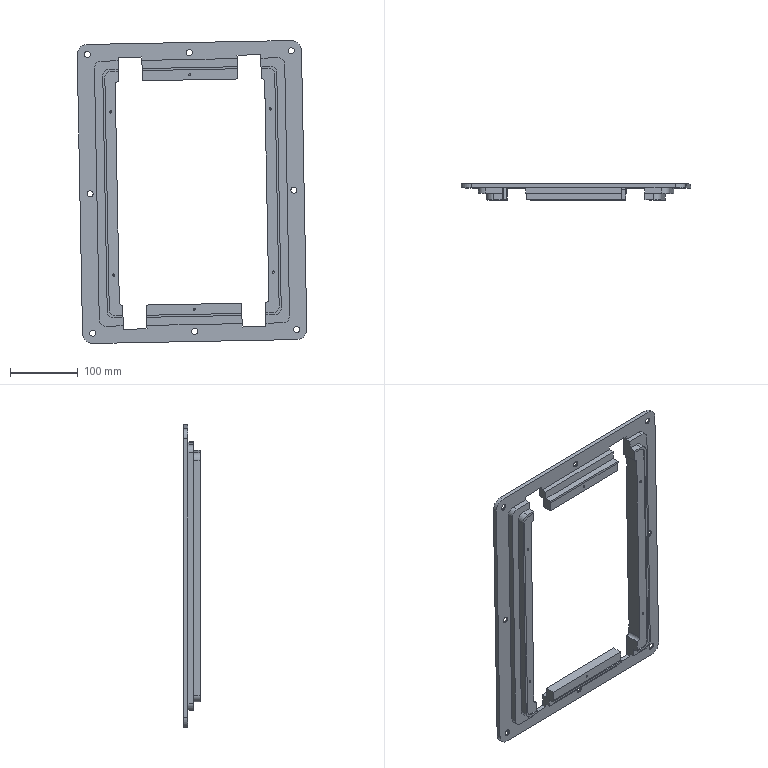Component | SolidWorks | 15BrushPlateThickInnerFrameOneOutOfTwo-1 | 1 solid | 141 faces | box 337.75 x 24 x 445.64 mm | volume 782663 mm3 | plane 63 | cylinder 50 | cone 28 | commonest cylinder face diameters 9 x16 3.3 x12 20 x12 10 x4 30 x4 12.125 x2 | material A3 Steel
build123d program:
from build123d import *

# Parameters (mm, degrees)
BOSS_EXTRUDE1_DEPTH                                  = 6
BOSS_EXTRUDE2_DEPTH                                  = 18
CUT_EXTRUDE1_DEPTH                                   = 277.045
CUT_EXTRUDE2_DEPTH                                   = 1.5
HOLE_SIZE_ACCORDING_TO_TYPE_OF_HEXAGON_S_D           = 9
HOLE_SIZE_ACCORDING_TO_TYPE_OF_HEXAGON_S_CSINK_D     = 17.6
HOLE_SIZE_ACCORDING_TO_TYPE_OF_HEXAGON_S_CSINK_ANGLE = 90
M4_TAPPED_HOLE1_D                                    = 3.3
M4_TAPPED_HOLE1_DEPTH                                = 8.1
M4_TAPPED_HOLE1_TIP                                  = 0.9914
CUT_EXTRUDE3_START                                   = -10
CUT_EXTRUDE3_DEPTH                                   = 10
SKETCH13_W                                           = 35
SKETCH13_H                                           = 35
CUT_EXTRUDE4_DEPTH                                   = 277.045
MIRROR2_COPY_1_SKETCH_W                              = 35
MIRROR2_COPY_1_SKETCH_H                              = 35
MIRROR2_COPY_1_DEPTH                                 = 277.045
SKETCH14_W                                           = 16
SKETCH14_H                                           = 140
CUT_EXTRUDE5_DEPTH                                   = 8
CUT_EXTRUDE6_REACH                                   = 399.336
SKETCH15_R                                           = 6.062


with BuildPart() as part:
    # Sketch1 → Boss-Extrude1 (new body)
    with BuildSketch(Plane.XY):
        with BuildLine():
            Line((-205, -165), (205, -165))
            ThreePointArc((205, -165), (215.607, -160.607), (220, -150))
            Line((220, -150), (220, 150))
            ThreePointArc((220, 150), (215.607, 160.607), (205, 165))
            Line((205, 165), (-205, 165))
            ThreePointArc((-205, 165), (-215.607, 160.607), (-220, 150))
            Line((-220, 150), (-220, -150))
            ThreePointArc((-220, -150), (-215.607, -160.607), (-205, -165))
        make_face()
    extrude(amount=-BOSS_EXTRUDE1_DEPTH)

    # Sketch2 → Boss-Extrude2 (add)
    with BuildSketch(Plane(origin=(0, 0, -6), x_dir=(-1, 0, 0), z_dir=(0, 0, -1))):
        with BuildLine():
            Line((-185, -140), (185, -140))
            ThreePointArc((185, -140), (192.071, -137.071), (195, -130))
            Line((195, -130), (195, 130))
            ThreePointArc((195, 130), (192.071, 137.071), (185, 140))
            Line((185, 140), (-185, 140))
            ThreePointArc((-185, 140), (-192.071, 137.071), (-195, 130))
            Line((-195, 130), (-195, -130))
            ThreePointArc((-195, -130), (-192.071, -137.071), (-185, -140))
        make_face()
    extrude(amount=BOSS_EXTRUDE2_DEPTH)

    # Sketch3 → Cut-Extrude1 (cut, through all)
    with BuildSketch(Plane.XY):
        with BuildLine():
            Line((-160, -110), (160, -110))
            ThreePointArc((160, -110), (163.536, -108.536), (165, -105))
            Line((165, -105), (165, 105))
            ThreePointArc((165, 105), (163.536, 108.536), (160, 110))
            Line((160, 110), (-160, 110))
            ThreePointArc((-160, 110), (-163.536, 108.536), (-165, 105))
            Line((-165, 105), (-165, -105))
            ThreePointArc((-165, -105), (-163.536, -108.536), (-160, -110))
        make_face()
    extrude(amount=-CUT_EXTRUDE1_DEPTH, mode=Mode.SUBTRACT)

    # Sketch4 → Cut-Extrude2 (cut)
    with BuildSketch(Plane.XY.offset(-24)):
        with BuildLine():
            Line((-170, -125), (170, -125))
            ThreePointArc((170, -125), (177.071, -122.071), (180, -115))
            Line((180, -115), (180, 115))
            ThreePointArc((180, 115), (177.071, 122.071), (170, 125))
            Line((170, 125), (-170, 125))
            ThreePointArc((-170, 125), (-177.071, 122.071), (-180, 115))
            Line((-180, 115), (-180, -115))
            ThreePointArc((-180, -115), (-177.071, -122.071), (-170, -125))
        make_face()
    extrude(amount=CUT_EXTRUDE2_DEPTH, mode=Mode.SUBTRACT)

    # Hole Size_According to_Type of Hexagon S (through all)
    with Locations(Plane(origin=(-205, 150, 0), x_dir=(1, 0, 0), z_dir=(0, 0, 1))):
        with Locations((0, 0), (0, -300), (410, -300), (410, 0), (410, -150), (205, 0), (0, -150), (205, -300)):
            CounterSinkHole(HOLE_SIZE_ACCORDING_TO_TYPE_OF_HEXAGON_S_D / 2, HOLE_SIZE_ACCORDING_TO_TYPE_OF_HEXAGON_S_CSINK_D / 2, counter_sink_angle=HOLE_SIZE_ACCORDING_TO_TYPE_OF_HEXAGON_S_CSINK_ANGLE)

    # M4 Tapped Hole1
    with Locations(Plane(origin=(172.5, 0, -22.5), x_dir=(-1, 0, 0), z_dir=(0, 0, -1))):
        with Locations((0, 0), (345, 0), (292.5, 117.5), (52.5, 117.5), (292.5, -117.5), (52.5, -117.5)):
            Hole(M4_TAPPED_HOLE1_D / 2, depth=M4_TAPPED_HOLE1_DEPTH)
            with Locations((0, 0, -(M4_TAPPED_HOLE1_DEPTH + M4_TAPPED_HOLE1_TIP / 2))):  # 118° drill point
                Cone(0, M4_TAPPED_HOLE1_D / 2, M4_TAPPED_HOLE1_TIP, mode=Mode.SUBTRACT)

    # Sketch12 → Cut-Extrude3 (cut)
    with BuildSketch(Plane(origin=(0, 0, -24), x_dir=(-1, 0, 0), z_dir=(0, 0, -1)).offset(CUT_EXTRUDE3_START)):
        with BuildLine():
            Line((185, 140), (-185, 140))
            ThreePointArc((-185, 140), (-192.071, 137.071), (-195, 130))
            Line((-195, 130), (-195, -130))
            ThreePointArc((-195, -130), (-192.071, -137.071), (-185, -140))
            Line((-185, -140), (185, -140))
            ThreePointArc((185, -140), (192.071, -137.071), (195, -130))
            Line((195, -130), (195, 130))
            ThreePointArc((195, 130), (192.071, 137.071), (185, 140))
        make_face()
        with BuildLine():
            Line((-173, -128), (173, -128))
            ThreePointArc((173, -128), (180.071, -125.071), (183, -118))
            Line((183, -118), (183, 118))
            ThreePointArc((183, 118), (180.071, 125.071), (173, 128))
            Line((173, 128), (-173, 128))
            ThreePointArc((-173, 128), (-180.071, 125.071), (-183, 118))
            Line((-183, 118), (-183, -118))
            ThreePointArc((-183, -118), (-180.071, -125.071), (-173, -128))
        make_face(mode=Mode.SUBTRACT)
    extrude(amount=CUT_EXTRUDE3_DEPTH, mode=Mode.SUBTRACT)

    # Sketch13 → Cut-Extrude4 (cut, through all)
    with BuildSketch(Plane.XY):
        with Locations((-182.5, 87.5)):
            Rectangle(SKETCH13_W, SKETCH13_H)
    cut_extrude4 = extrude(amount=-CUT_EXTRUDE4_DEPTH, mode=Mode.SUBTRACT)

    # Mirror1: Cut-Extrude4 across plane
    add(cut_extrude4.mirror(Plane.ZX), mode=Mode.SUBTRACT)

    # Mirror2: Cut-Extrude4 across plane
    add(cut_extrude4.mirror(Plane(origin=(0, 0, 0), x_dir=(0, 0, 1), z_dir=(1, 0, 0))), mode=Mode.SUBTRACT)

    # Mirror2 copy 1 sketch → Mirror2 copy 1 (cut, through all)
    with BuildSketch(Plane(origin=(0, 0, 0), x_dir=(-1, 0, 0), z_dir=(0, 0, 1))):
        with Locations((-182.5, 87.5)):
            Rectangle(MIRROR2_COPY_1_SKETCH_W, MIRROR2_COPY_1_SKETCH_H)
    extrude(amount=-MIRROR2_COPY_1_DEPTH, mode=Mode.SUBTRACT)

    # Sketch14 → Cut-Extrude5 (cut)
    with BuildSketch(Plane.XY):
        with Locations((-173, 0)):
            Rectangle(SKETCH14_W, SKETCH14_H)
    cut_extrude5 = extrude(amount=-CUT_EXTRUDE5_DEPTH, mode=Mode.SUBTRACT)

    # Mirror3: Cut-Extrude5 across plane
    add(cut_extrude5.mirror(Plane(origin=(0, 0, 0), x_dir=(0, 0, 1), z_dir=(1, 0, 0))), mode=Mode.SUBTRACT)

    # Sketch15 → Cut-Extrude6 (cut, up to next)
    with BuildSketch(Plane(origin=(0, 165, 0), x_dir=(1, 0, 0), z_dir=(0, 1, 0)), mode=Mode.PRIVATE) as cut_extrude6_sk1:
        with Locations((-143.5, -4.062)):
            Circle(SKETCH15_R)
    cut_extrude6_tool1 = extrude(cut_extrude6_sk1.sketch, amount=-CUT_EXTRUDE6_REACH, mode=Mode.PRIVATE) & part.part
    cut_extrude6 = cut_extrude6_tool1.solids().sort_by_distance((-143.5, 165, 4.062))[0]
    add(cut_extrude6, mode=Mode.SUBTRACT)

    # Mirror4: Cut-Extrude6 across plane
    add(cut_extrude6.mirror(Plane(origin=(0, 0, 0), x_dir=(0, 0, 1), z_dir=(1, 0, 0))), mode=Mode.SUBTRACT)


solid = part.part

# Placed as in the assembly
solid = solid.moved(Location((222.878, -1615.522, 2069.362), (-90, 0, -91.091)))